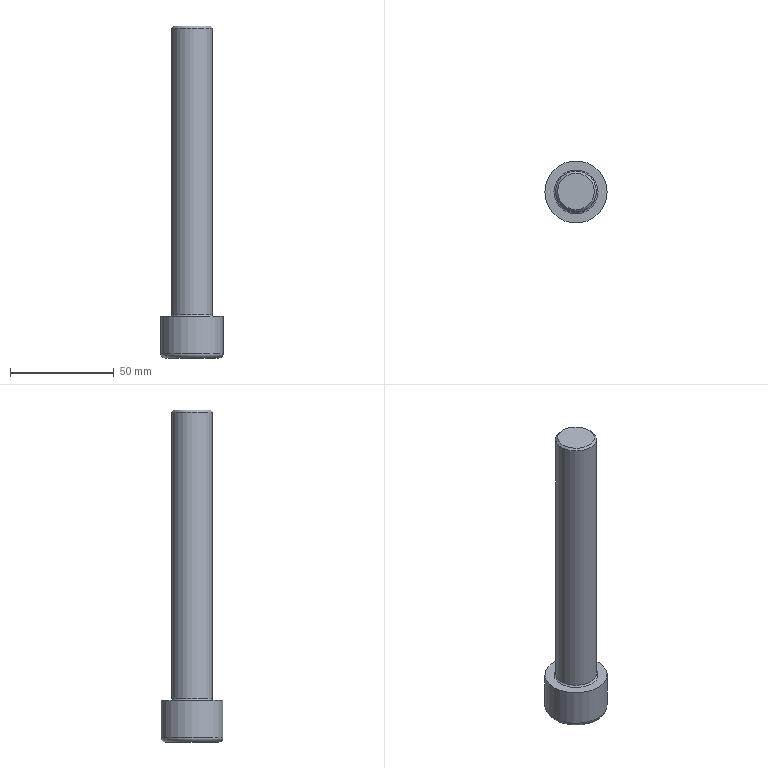Component | NX | GB-T70_1-2000_M20X140 | 1 solid | 27 faces | volume 53138 mm3 | plane 15 | cone 8 | cylinder 2 | torus 2 | commonest cylinder face diameters 19.623 x1 30 x1